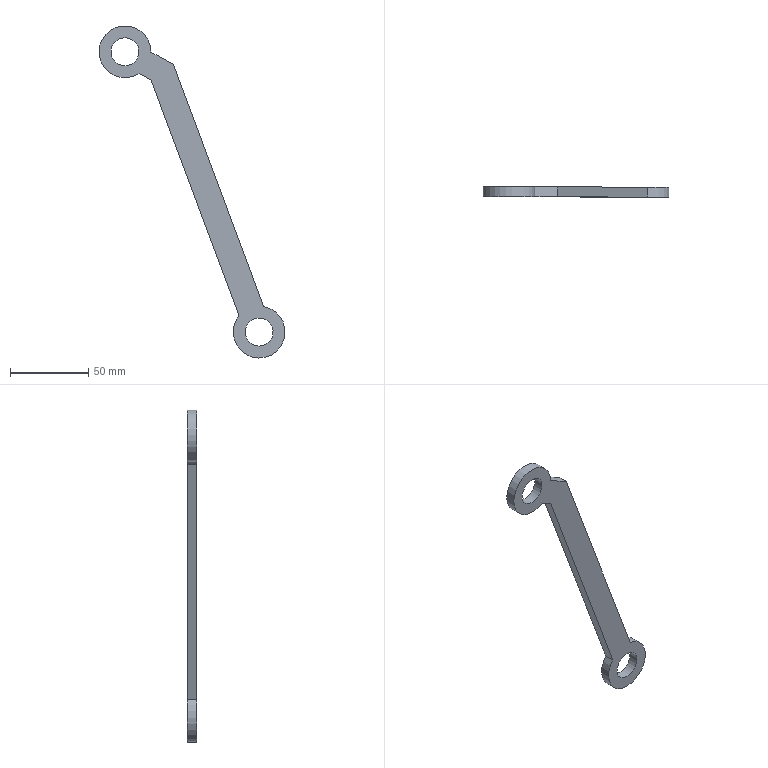Component | NX | LINK | 1 solid | 10 faces | box 118.49 x 6.35 x 211.58 mm | volume 25994 mm3 | plane 6 | cylinder 4 | commonest cylinder face diameters 33.02 x2 17.78 x2
STEP:
#1=CARTESIAN_POINT('',(0.,0.,0.));
#2=DIRECTION('',(0.,0.,1.));
#3=DIRECTION('',(1.,0.,0.));
#4=AXIS2_PLACEMENT_3D('',#1,#2,#3);
#5=CARTESIAN_POINT('',(88.37,21.5,328.882));
#6=VERTEX_POINT('',#5);
#7=CARTESIAN_POINT('',(72.634,21.5,323.014));
#8=VERTEX_POINT('',#7);
#9=CARTESIAN_POINT('',(85.469,21.5,312.629));
#10=DIRECTION('',(0.,1.,0.));
#11=DIRECTION('',(0.937,0.,0.3494));
#12=AXIS2_PLACEMENT_3D('',#9,#10,#11);
#13=CIRCLE('',#12,16.51);
#14=CARTESIAN_POINT('',(85.469,15.15,312.629));
#15=DIRECTION('',(0.,1.,0.));
#16=DIRECTION('',(-0.937,0.,-0.3494));
#17=AXIS2_PLACEMENT_3D('',#14,#15,#16);
#18=CYLINDRICAL_SURFACE('',#17,16.51);
#19=CARTESIAN_POINT('',(-3.142,6.35));
#20=DIRECTION('',(1.,0.));
#21=VECTOR('',#20,1.);
#22=LINE('',#19,#21);
#23=(GEOMETRIC_REPRESENTATION_CONTEXT(2)PARAMETRIC_REPRESENTATION_CONTEXT()REPRESENTATION_CONTEXT('',''));
#24=DEFINITIONAL_REPRESENTATION('',(#22),#23);
#25=PCURVE('',#18,#24);
#26=CARTESIAN_POINT('',(85.469,21.5,312.629));
#27=DIRECTION('',(0.,1.,0.));
#28=DIRECTION('',(-0.937,0.,-0.3494));
#29=AXIS2_PLACEMENT_3D('',#26,#27,#28);
#30=PLANE('',#29);
#31=CARTESIAN_POINT('',(0.,0.));
#32=DIRECTION('',(-1.,0.));
#33=AXIS2_PLACEMENT_2D('',#31,#32);
#34=CIRCLE('',#33,16.51);
#35=(GEOMETRIC_REPRESENTATION_CONTEXT(2)PARAMETRIC_REPRESENTATION_CONTEXT()REPRESENTATION_CONTEXT('',''));
#36=DEFINITIONAL_REPRESENTATION('',(#34),#35);
#37=PCURVE('',#30,#36);
#38=SURFACE_CURVE('',#13,(#25,#37),.PCURVE_S1.);
#39=EDGE_CURVE('',#6,#8,#38,.T.);
#40=ORIENTED_EDGE('',*,*,#39,.F.);
#41=CARTESIAN_POINT('',(88.37,15.15,328.882));
#42=VERTEX_POINT('',#41);
#43=CARTESIAN_POINT('',(88.37,15.15,328.882));
#44=DIRECTION('',(0.,1.,0.));
#45=VECTOR('',#44,1.);
#46=LINE('',#43,#45);
#47=CARTESIAN_POINT('',(2.104,0.));
#48=DIRECTION('',(0.,1.));
#49=VECTOR('',#48,1.);
#50=LINE('',#47,#49);
#51=(GEOMETRIC_REPRESENTATION_CONTEXT(2)PARAMETRIC_REPRESENTATION_CONTEXT()REPRESENTATION_CONTEXT('',''));
#52=DEFINITIONAL_REPRESENTATION('',(#50),#51);
#53=PCURVE('',#18,#52);
#54=CARTESIAN_POINT('',(30.849,15.15,483.124));
#55=DIRECTION('',(0.937,0.,0.3494));
#56=DIRECTION('',(-0.3494,0.,0.937));
#57=AXIS2_PLACEMENT_3D('',#54,#55,#56);
#58=PLANE('',#57);
#59=CARTESIAN_POINT('',(-164.619,0.));
#60=DIRECTION('',(0.,-1.));
#61=VECTOR('',#60,1.);
#62=LINE('',#59,#61);
#63=(GEOMETRIC_REPRESENTATION_CONTEXT(2)PARAMETRIC_REPRESENTATION_CONTEXT()REPRESENTATION_CONTEXT('',''));
#64=DEFINITIONAL_REPRESENTATION('',(#62),#63);
#65=PCURVE('',#58,#64);
#66=SURFACE_CURVE('',#46,(#53,#65),.PCURVE_S1.);
#67=EDGE_CURVE('',#42,#6,#66,.T.);
#68=ORIENTED_EDGE('',*,*,#67,.F.);
#69=CARTESIAN_POINT('',(72.634,15.15,323.014));
#70=VERTEX_POINT('',#69);
#71=CARTESIAN_POINT('',(85.469,15.15,312.629));
#72=DIRECTION('',(0.,1.,0.));
#73=DIRECTION('',(0.937,0.,0.3494));
#74=AXIS2_PLACEMENT_3D('',#71,#72,#73);
#75=CIRCLE('',#74,16.51);
#76=CARTESIAN_POINT('',(-3.142,0.));
#77=DIRECTION('',(1.,0.));
#78=VECTOR('',#77,1.);
#79=LINE('',#76,#78);
#80=(GEOMETRIC_REPRESENTATION_CONTEXT(2)PARAMETRIC_REPRESENTATION_CONTEXT()REPRESENTATION_CONTEXT('',''));
#81=DEFINITIONAL_REPRESENTATION('',(#79),#80);
#82=PCURVE('',#18,#81);
#83=CARTESIAN_POINT('',(85.469,15.15,312.629));
#84=DIRECTION('',(0.,1.,0.));
#85=DIRECTION('',(-0.937,0.,-0.3494));
#86=AXIS2_PLACEMENT_3D('',#83,#84,#85);
#87=PLANE('',#86);
#88=CARTESIAN_POINT('',(0.,0.));
#89=DIRECTION('',(-1.,0.));
#90=AXIS2_PLACEMENT_2D('',#88,#89);
#91=CIRCLE('',#90,16.51);
#92=(GEOMETRIC_REPRESENTATION_CONTEXT(2)PARAMETRIC_REPRESENTATION_CONTEXT()REPRESENTATION_CONTEXT('',''));
#93=DEFINITIONAL_REPRESENTATION('',(#91),#92);
#94=PCURVE('',#87,#93);
#95=SURFACE_CURVE('',#75,(#82,#94),.PCURVE_S1.);
#96=EDGE_CURVE('',#42,#70,#95,.T.);
#97=ORIENTED_EDGE('',*,*,#96,.T.);
#98=CARTESIAN_POINT('',(72.634,15.15,323.014));
#99=DIRECTION('',(0.,1.,0.));
#100=VECTOR('',#99,1.);
#101=LINE('',#98,#100);
#102=CARTESIAN_POINT('',(7.32,0.));
#103=DIRECTION('',(0.,1.));
#104=VECTOR('',#103,1.);
#105=LINE('',#102,#104);
#106=(GEOMETRIC_REPRESENTATION_CONTEXT(2)PARAMETRIC_REPRESENTATION_CONTEXT()REPRESENTATION_CONTEXT('',''));
#107=DEFINITIONAL_REPRESENTATION('',(#105),#106);
#108=PCURVE('',#18,#107);
#109=CARTESIAN_POINT('',(72.634,15.15,323.014));
#110=DIRECTION('',(-0.937,0.,-0.3494));
#111=DIRECTION('',(0.3494,0.,-0.937));
#112=AXIS2_PLACEMENT_3D('',#109,#110,#111);
#113=PLANE('',#112);
#114=CARTESIAN_POINT('',(0.,0.));
#115=DIRECTION('',(0.,-1.));
#116=VECTOR('',#115,1.);
#117=LINE('',#114,#116);
#118=(GEOMETRIC_REPRESENTATION_CONTEXT(2)PARAMETRIC_REPRESENTATION_CONTEXT()REPRESENTATION_CONTEXT('',''));
#119=DEFINITIONAL_REPRESENTATION('',(#117),#118);
#120=PCURVE('',#113,#119);
#121=SURFACE_CURVE('',#101,(#108,#120),.PCURVE_S1.);
#122=EDGE_CURVE('',#70,#8,#121,.T.);
#123=ORIENTED_EDGE('',*,*,#122,.T.);
#124=EDGE_LOOP('',(#40,#68,#97,#123));
#125=FACE_BOUND('',#124,.T.);
#126=ADVANCED_FACE('',(#125),#18,.T.);
#127=CARTESIAN_POINT('',(16.679,21.5,473.058));
#128=VERTEX_POINT('',#127);
#129=CARTESIAN_POINT('',(72.634,21.5,323.014));
#130=DIRECTION('',(-0.3494,0.,0.937));
#131=VECTOR('',#130,1.);
#132=LINE('',#129,#131);
#133=CARTESIAN_POINT('',(0.,-6.35));
#134=DIRECTION('',(-1.,0.));
#135=VECTOR('',#134,1.);
#136=LINE('',#133,#135);
#137=(GEOMETRIC_REPRESENTATION_CONTEXT(2)PARAMETRIC_REPRESENTATION_CONTEXT()REPRESENTATION_CONTEXT('',''));
#138=DEFINITIONAL_REPRESENTATION('',(#136),#137);
#139=PCURVE('',#113,#138);
#140=CARTESIAN_POINT('',(8.397,14.215));
#141=DIRECTION('',(0.,1.));
#142=VECTOR('',#141,1.);
#143=LINE('',#140,#142);
#144=(GEOMETRIC_REPRESENTATION_CONTEXT(2)PARAMETRIC_REPRESENTATION_CONTEXT()REPRESENTATION_CONTEXT('',''));
#145=DEFINITIONAL_REPRESENTATION('',(#143),#144);
#146=PCURVE('',#30,#145);
#147=SURFACE_CURVE('',#132,(#139,#146),.PCURVE_S1.);
#148=EDGE_CURVE('',#8,#128,#147,.T.);
#149=ORIENTED_EDGE('',*,*,#148,.F.);
#150=ORIENTED_EDGE('',*,*,#122,.F.);
#151=CARTESIAN_POINT('',(16.679,15.15,473.058));
#152=VERTEX_POINT('',#151);
#153=CARTESIAN_POINT('',(72.634,15.15,323.014));
#154=DIRECTION('',(-0.3494,0.,0.937));
#155=VECTOR('',#154,1.);
#156=LINE('',#153,#155);
#157=CARTESIAN_POINT('',(0.,0.));
#158=DIRECTION('',(-1.,0.));
#159=VECTOR('',#158,1.);
#160=LINE('',#157,#159);
#161=(GEOMETRIC_REPRESENTATION_CONTEXT(2)PARAMETRIC_REPRESENTATION_CONTEXT()REPRESENTATION_CONTEXT('',''));
#162=DEFINITIONAL_REPRESENTATION('',(#160),#161);
#163=PCURVE('',#113,#162);
#164=CARTESIAN_POINT('',(8.397,14.215));
#165=DIRECTION('',(0.,1.));
#166=VECTOR('',#165,1.);
#167=LINE('',#164,#166);
#168=(GEOMETRIC_REPRESENTATION_CONTEXT(2)PARAMETRIC_REPRESENTATION_CONTEXT()REPRESENTATION_CONTEXT('',''));
#169=DEFINITIONAL_REPRESENTATION('',(#167),#168);
#170=PCURVE('',#87,#169);
#171=SURFACE_CURVE('',#156,(#163,#170),.PCURVE_S1.);
#172=EDGE_CURVE('',#70,#152,#171,.T.);
#173=ORIENTED_EDGE('',*,*,#172,.T.);
#174=CARTESIAN_POINT('',(16.679,15.15,473.058));
#175=DIRECTION('',(0.,1.,0.));
#176=VECTOR('',#175,1.);
#177=LINE('',#174,#176);
#178=CARTESIAN_POINT('',(-160.139,0.));
#179=DIRECTION('',(0.,-1.));
#180=VECTOR('',#179,1.);
#181=LINE('',#178,#180);
#182=(GEOMETRIC_REPRESENTATION_CONTEXT(2)PARAMETRIC_REPRESENTATION_CONTEXT()REPRESENTATION_CONTEXT('',''));
#183=DEFINITIONAL_REPRESENTATION('',(#181),#182);
#184=PCURVE('',#113,#183);
#185=CARTESIAN_POINT('',(16.679,15.15,473.058));
#186=DIRECTION('',(-0.4827,0.,-0.8758));
#187=DIRECTION('',(0.8758,0.,-0.4827));
#188=AXIS2_PLACEMENT_3D('',#185,#186,#187);
#189=PLANE('',#188);
#190=CARTESIAN_POINT('',(0.,0.));
#191=DIRECTION('',(0.,-1.));
#192=VECTOR('',#191,1.);
#193=LINE('',#190,#192);
#194=(GEOMETRIC_REPRESENTATION_CONTEXT(2)PARAMETRIC_REPRESENTATION_CONTEXT()REPRESENTATION_CONTEXT('',''));
#195=DEFINITIONAL_REPRESENTATION('',(#193),#194);
#196=PCURVE('',#189,#195);
#197=SURFACE_CURVE('',#177,(#184,#196),.PCURVE_S1.);
#198=EDGE_CURVE('',#152,#128,#197,.T.);
#199=ORIENTED_EDGE('',*,*,#198,.T.);
#200=EDGE_LOOP('',(#149,#150,#173,#199));
#201=FACE_BOUND('',#200,.T.);
#202=ADVANCED_FACE('',(#201),#113,.T.);
#203=CARTESIAN_POINT('',(8.952,21.5,477.318));
#204=VERTEX_POINT('',#203);
#205=CARTESIAN_POINT('',(16.679,21.5,473.058));
#206=DIRECTION('',(-0.8758,0.,0.4827));
#207=VECTOR('',#206,1.);
#208=LINE('',#205,#207);
#209=CARTESIAN_POINT('',(0.,-6.35));
#210=DIRECTION('',(-1.,0.));
#211=VECTOR('',#210,1.);
#212=LINE('',#209,#211);
#213=(GEOMETRIC_REPRESENTATION_CONTEXT(2)PARAMETRIC_REPRESENTATION_CONTEXT()REPRESENTATION_CONTEXT('',''));
#214=DEFINITIONAL_REPRESENTATION('',(#212),#213);
#215=PCURVE('',#189,#214);
#216=CARTESIAN_POINT('',(8.397,174.354));
#217=DIRECTION('',(0.6519,0.7583));
#218=VECTOR('',#217,1.);
#219=LINE('',#216,#218);
#220=(GEOMETRIC_REPRESENTATION_CONTEXT(2)PARAMETRIC_REPRESENTATION_CONTEXT()REPRESENTATION_CONTEXT('',''));
#221=DEFINITIONAL_REPRESENTATION('',(#219),#220);
#222=PCURVE('',#30,#221);
#223=SURFACE_CURVE('',#208,(#215,#222),.PCURVE_S1.);
#224=EDGE_CURVE('',#128,#204,#223,.T.);
#225=ORIENTED_EDGE('',*,*,#224,.F.);
#226=ORIENTED_EDGE('',*,*,#198,.F.);
#227=CARTESIAN_POINT('',(8.952,15.15,477.318));
#228=VERTEX_POINT('',#227);
#229=CARTESIAN_POINT('',(16.679,15.15,473.058));
#230=DIRECTION('',(-0.8758,0.,0.4827));
#231=VECTOR('',#230,1.);
#232=LINE('',#229,#231);
#233=CARTESIAN_POINT('',(0.,0.));
#234=DIRECTION('',(-1.,0.));
#235=VECTOR('',#234,1.);
#236=LINE('',#233,#235);
#237=(GEOMETRIC_REPRESENTATION_CONTEXT(2)PARAMETRIC_REPRESENTATION_CONTEXT()REPRESENTATION_CONTEXT('',''));
#238=DEFINITIONAL_REPRESENTATION('',(#236),#237);
#239=PCURVE('',#189,#238);
#240=CARTESIAN_POINT('',(8.397,174.354));
#241=DIRECTION('',(0.6519,0.7583));
#242=VECTOR('',#241,1.);
#243=LINE('',#240,#242);
#244=(GEOMETRIC_REPRESENTATION_CONTEXT(2)PARAMETRIC_REPRESENTATION_CONTEXT()REPRESENTATION_CONTEXT('',''));
#245=DEFINITIONAL_REPRESENTATION('',(#243),#244);
#246=PCURVE('',#87,#245);
#247=SURFACE_CURVE('',#232,(#239,#246),.PCURVE_S1.);
#248=EDGE_CURVE('',#152,#228,#247,.T.);
#249=ORIENTED_EDGE('',*,*,#248,.T.);
#250=CARTESIAN_POINT('',(8.952,15.15,477.318));
#251=DIRECTION('',(0.,1.,0.));
#252=VECTOR('',#251,1.);
#253=LINE('',#250,#252);
#254=CARTESIAN_POINT('',(-8.823,0.));
#255=DIRECTION('',(0.,-1.));
#256=VECTOR('',#255,1.);
#257=LINE('',#254,#256);
#258=(GEOMETRIC_REPRESENTATION_CONTEXT(2)PARAMETRIC_REPRESENTATION_CONTEXT()REPRESENTATION_CONTEXT('',''));
#259=DEFINITIONAL_REPRESENTATION('',(#257),#258);
#260=PCURVE('',#189,#259);
#261=CARTESIAN_POINT('',(0.,15.15,491.19));
#262=DIRECTION('',(0.,1.,0.));
#263=DIRECTION('',(-0.937,0.,-0.3494));
#264=AXIS2_PLACEMENT_3D('',#261,#262,#263);
#265=CYLINDRICAL_SURFACE('',#264,16.51);
#266=CARTESIAN_POINT('',(-1.787,0.));
#267=DIRECTION('',(0.,1.));
#268=VECTOR('',#267,1.);
#269=LINE('',#266,#268);
#270=(GEOMETRIC_REPRESENTATION_CONTEXT(2)PARAMETRIC_REPRESENTATION_CONTEXT()REPRESENTATION_CONTEXT('',''));
#271=DEFINITIONAL_REPRESENTATION('',(#269),#270);
#272=PCURVE('',#265,#271);
#273=SURFACE_CURVE('',#253,(#260,#272),.PCURVE_S1.);
#274=EDGE_CURVE('',#228,#204,#273,.T.);
#275=ORIENTED_EDGE('',*,*,#274,.T.);
#276=EDGE_LOOP('',(#225,#226,#249,#275));
#277=FACE_BOUND('',#276,.T.);
#278=ADVANCED_FACE('',(#277),#189,.T.);
#279=CARTESIAN_POINT('',(16.509,21.5,491.028));
#280=VERTEX_POINT('',#279);
#281=CARTESIAN_POINT('',(0.,21.5,491.19));
#282=DIRECTION('',(0.,1.,0.));
#283=DIRECTION('',(0.937,0.,0.3494));
#284=AXIS2_PLACEMENT_3D('',#281,#282,#283);
#285=CIRCLE('',#284,16.51);
#286=CARTESIAN_POINT('',(-3.142,6.35));
#287=DIRECTION('',(1.,0.));
#288=VECTOR('',#287,1.);
#289=LINE('',#286,#288);
#290=(GEOMETRIC_REPRESENTATION_CONTEXT(2)PARAMETRIC_REPRESENTATION_CONTEXT()REPRESENTATION_CONTEXT('',''));
#291=DEFINITIONAL_REPRESENTATION('',(#289),#290);
#292=PCURVE('',#265,#291);
#293=CARTESIAN_POINT('',(17.689,197.171));
#294=DIRECTION('',(-1.,0.));
#295=AXIS2_PLACEMENT_2D('',#293,#294);
#296=CIRCLE('',#295,16.51);
#297=(GEOMETRIC_REPRESENTATION_CONTEXT(2)PARAMETRIC_REPRESENTATION_CONTEXT()REPRESENTATION_CONTEXT('',''));
#298=DEFINITIONAL_REPRESENTATION('',(#296),#297);
#299=PCURVE('',#30,#298);
#300=SURFACE_CURVE('',#285,(#292,#299),.PCURVE_S1.);
#301=EDGE_CURVE('',#204,#280,#300,.T.);
#302=ORIENTED_EDGE('',*,*,#301,.F.);
#303=ORIENTED_EDGE('',*,*,#274,.F.);
#304=CARTESIAN_POINT('',(16.509,15.15,491.028));
#305=VERTEX_POINT('',#304);
#306=CARTESIAN_POINT('',(0.,15.15,491.19));
#307=DIRECTION('',(0.,1.,0.));
#308=DIRECTION('',(0.937,0.,0.3494));
#309=AXIS2_PLACEMENT_3D('',#306,#307,#308);
#310=CIRCLE('',#309,16.51);
#311=CARTESIAN_POINT('',(-3.142,0.));
#312=DIRECTION('',(1.,0.));
#313=VECTOR('',#312,1.);
#314=LINE('',#311,#313);
#315=(GEOMETRIC_REPRESENTATION_CONTEXT(2)PARAMETRIC_REPRESENTATION_CONTEXT()REPRESENTATION_CONTEXT('',''));
#316=DEFINITIONAL_REPRESENTATION('',(#314),#315);
#317=PCURVE('',#265,#316);
#318=CARTESIAN_POINT('',(17.689,197.171));
#319=DIRECTION('',(-1.,0.));
#320=AXIS2_PLACEMENT_2D('',#318,#319);
#321=CIRCLE('',#320,16.51);
#322=(GEOMETRIC_REPRESENTATION_CONTEXT(2)PARAMETRIC_REPRESENTATION_CONTEXT()REPRESENTATION_CONTEXT('',''));
#323=DEFINITIONAL_REPRESENTATION('',(#321),#322);
#324=PCURVE('',#87,#323);
#325=SURFACE_CURVE('',#310,(#317,#324),.PCURVE_S1.);
#326=EDGE_CURVE('',#228,#305,#325,.T.);
#327=ORIENTED_EDGE('',*,*,#326,.T.);
#328=CARTESIAN_POINT('',(16.509,15.15,491.028));
#329=DIRECTION('',(0.,1.,0.));
#330=VECTOR('',#329,1.);
#331=LINE('',#328,#330);
#332=CARTESIAN_POINT('',(3.508,0.));
#333=DIRECTION('',(0.,1.));
#334=VECTOR('',#333,1.);
#335=LINE('',#332,#334);
#336=(GEOMETRIC_REPRESENTATION_CONTEXT(2)PARAMETRIC_REPRESENTATION_CONTEXT()REPRESENTATION_CONTEXT('',''));
#337=DEFINITIONAL_REPRESENTATION('',(#335),#336);
#338=PCURVE('',#265,#337);
#339=CARTESIAN_POINT('',(16.509,15.15,491.028));
#340=DIRECTION('',(0.4827,0.,0.8758));
#341=DIRECTION('',(-0.8758,0.,0.4827));
#342=AXIS2_PLACEMENT_3D('',#339,#340,#341);
#343=PLANE('',#342);
#344=CARTESIAN_POINT('',(0.,0.));
#345=DIRECTION('',(0.,-1.));
#346=VECTOR('',#345,1.);
#347=LINE('',#344,#346);
#348=(GEOMETRIC_REPRESENTATION_CONTEXT(2)PARAMETRIC_REPRESENTATION_CONTEXT()REPRESENTATION_CONTEXT('',''));
#349=DEFINITIONAL_REPRESENTATION('',(#347),#348);
#350=PCURVE('',#343,#349);
#351=SURFACE_CURVE('',#331,(#338,#350),.PCURVE_S1.);
#352=EDGE_CURVE('',#305,#280,#351,.T.);
#353=ORIENTED_EDGE('',*,*,#352,.T.);
#354=EDGE_LOOP('',(#302,#303,#327,#353));
#355=FACE_BOUND('',#354,.T.);
#356=ADVANCED_FACE('',(#355),#265,.T.);
#357=CARTESIAN_POINT('',(30.849,21.5,483.124));
#358=VERTEX_POINT('',#357);
#359=CARTESIAN_POINT('',(16.509,21.5,491.028));
#360=DIRECTION('',(0.8758,0.,-0.4827));
#361=VECTOR('',#360,1.);
#362=LINE('',#359,#361);
#363=CARTESIAN_POINT('',(0.,-6.35));
#364=DIRECTION('',(-1.,0.));
#365=VECTOR('',#364,1.);
#366=LINE('',#363,#365);
#367=(GEOMETRIC_REPRESENTATION_CONTEXT(2)PARAMETRIC_REPRESENTATION_CONTEXT()REPRESENTATION_CONTEXT('',''));
#368=DEFINITIONAL_REPRESENTATION('',(#366),#367);
#369=PCURVE('',#343,#368);
#370=CARTESIAN_POINT('',(2.277,191.251));
#371=DIRECTION('',(-0.6519,-0.7583));
#372=VECTOR('',#371,1.);
#373=LINE('',#370,#372);
#374=(GEOMETRIC_REPRESENTATION_CONTEXT(2)PARAMETRIC_REPRESENTATION_CONTEXT()REPRESENTATION_CONTEXT('',''));
#375=DEFINITIONAL_REPRESENTATION('',(#373),#374);
#376=PCURVE('',#30,#375);
#377=SURFACE_CURVE('',#362,(#369,#376),.PCURVE_S1.);
#378=EDGE_CURVE('',#280,#358,#377,.T.);
#379=ORIENTED_EDGE('',*,*,#378,.F.);
#380=ORIENTED_EDGE('',*,*,#352,.F.);
#381=CARTESIAN_POINT('',(30.849,15.15,483.124));
#382=VERTEX_POINT('',#381);
#383=CARTESIAN_POINT('',(16.509,15.15,491.028));
#384=DIRECTION('',(0.8758,0.,-0.4827));
#385=VECTOR('',#384,1.);
#386=LINE('',#383,#385);
#387=CARTESIAN_POINT('',(0.,0.));
#388=DIRECTION('',(-1.,0.));
#389=VECTOR('',#388,1.);
#390=LINE('',#387,#389);
#391=(GEOMETRIC_REPRESENTATION_CONTEXT(2)PARAMETRIC_REPRESENTATION_CONTEXT()REPRESENTATION_CONTEXT('',''));
#392=DEFINITIONAL_REPRESENTATION('',(#390),#391);
#393=PCURVE('',#343,#392);
#394=CARTESIAN_POINT('',(2.277,191.251));
#395=DIRECTION('',(-0.6519,-0.7583));
#396=VECTOR('',#395,1.);
#397=LINE('',#394,#396);
#398=(GEOMETRIC_REPRESENTATION_CONTEXT(2)PARAMETRIC_REPRESENTATION_CONTEXT()REPRESENTATION_CONTEXT('',''));
#399=DEFINITIONAL_REPRESENTATION('',(#397),#398);
#400=PCURVE('',#87,#399);
#401=SURFACE_CURVE('',#386,(#393,#400),.PCURVE_S1.);
#402=EDGE_CURVE('',#305,#382,#401,.T.);
#403=ORIENTED_EDGE('',*,*,#402,.T.);
#404=CARTESIAN_POINT('',(30.849,15.15,483.124));
#405=DIRECTION('',(0.,1.,0.));
#406=VECTOR('',#405,1.);
#407=LINE('',#404,#406);
#408=CARTESIAN_POINT('',(-16.374,0.));
#409=DIRECTION('',(0.,-1.));
#410=VECTOR('',#409,1.);
#411=LINE('',#408,#410);
#412=(GEOMETRIC_REPRESENTATION_CONTEXT(2)PARAMETRIC_REPRESENTATION_CONTEXT()REPRESENTATION_CONTEXT('',''));
#413=DEFINITIONAL_REPRESENTATION('',(#411),#412);
#414=PCURVE('',#343,#413);
#415=CARTESIAN_POINT('',(0.,0.));
#416=DIRECTION('',(0.,-1.));
#417=VECTOR('',#416,1.);
#418=LINE('',#415,#417);
#419=(GEOMETRIC_REPRESENTATION_CONTEXT(2)PARAMETRIC_REPRESENTATION_CONTEXT()REPRESENTATION_CONTEXT('',''));
#420=DEFINITIONAL_REPRESENTATION('',(#418),#419);
#421=PCURVE('',#58,#420);
#422=SURFACE_CURVE('',#407,(#414,#421),.PCURVE_S1.);
#423=EDGE_CURVE('',#382,#358,#422,.T.);
#424=ORIENTED_EDGE('',*,*,#423,.T.);
#425=EDGE_LOOP('',(#379,#380,#403,#424));
#426=FACE_BOUND('',#425,.T.);
#427=ADVANCED_FACE('',(#426),#343,.T.);
#428=CARTESIAN_POINT('',(93.799,15.15,315.735));
#429=VERTEX_POINT('',#428);
#430=CARTESIAN_POINT('',(85.469,15.15,312.629));
#431=DIRECTION('',(0.,1.,0.));
#432=DIRECTION('',(0.937,0.,0.3494));
#433=AXIS2_PLACEMENT_3D('',#430,#431,#432);
#434=CIRCLE('',#433,8.89);
#435=CARTESIAN_POINT('',(85.469,15.15,312.629));
#436=DIRECTION('',(0.,1.,0.));
#437=DIRECTION('',(-0.937,0.,-0.3494));
#438=AXIS2_PLACEMENT_3D('',#435,#436,#437);
#439=CYLINDRICAL_SURFACE('',#438,8.89);
#440=CARTESIAN_POINT('',(3.142,0.));
#441=DIRECTION('',(1.,0.));
#442=VECTOR('',#441,1.);
#443=LINE('',#440,#442);
#444=(GEOMETRIC_REPRESENTATION_CONTEXT(2)PARAMETRIC_REPRESENTATION_CONTEXT()REPRESENTATION_CONTEXT('',''));
#445=DEFINITIONAL_REPRESENTATION('',(#443),#444);
#446=PCURVE('',#439,#445);
#447=CARTESIAN_POINT('',(0.,0.));
#448=DIRECTION('',(-1.,0.));
#449=AXIS2_PLACEMENT_2D('',#447,#448);
#450=CIRCLE('',#449,8.89);
#451=(GEOMETRIC_REPRESENTATION_CONTEXT(2)PARAMETRIC_REPRESENTATION_CONTEXT()REPRESENTATION_CONTEXT('',''));
#452=DEFINITIONAL_REPRESENTATION('',(#450),#451);
#453=PCURVE('',#87,#452);
#454=SURFACE_CURVE('',#434,(#446,#453),.PCURVE_S1.);
#455=EDGE_CURVE('',#429,#429,#454,.T.);
#456=ORIENTED_EDGE('',*,*,#455,.T.);
#457=CARTESIAN_POINT('',(93.799,21.5,315.735));
#458=VERTEX_POINT('',#457);
#459=CARTESIAN_POINT('',(93.799,15.15,315.735));
#460=CARTESIAN_POINT('',(93.799,21.5,315.735));
#461=B_SPLINE_CURVE_WITH_KNOTS('',1,(#459,#460),.UNSPECIFIED.,.F.,.F.,(2,2),(0.,6.35),.PIECEWISE_BEZIER_KNOTS.);
#462=CARTESIAN_POINT('',(9.425,0.));
#463=DIRECTION('',(0.,1.));
#464=VECTOR('',#463,1.);
#465=LINE('',#462,#464);
#466=(GEOMETRIC_REPRESENTATION_CONTEXT(2)PARAMETRIC_REPRESENTATION_CONTEXT()REPRESENTATION_CONTEXT('',''));
#467=DEFINITIONAL_REPRESENTATION('',(#465),#466);
#468=PCURVE('',#439,#467);
#469=CARTESIAN_POINT('',(3.142,0.));
#470=DIRECTION('',(0.,1.));
#471=VECTOR('',#470,1.);
#472=LINE('',#469,#471);
#473=(GEOMETRIC_REPRESENTATION_CONTEXT(2)PARAMETRIC_REPRESENTATION_CONTEXT()REPRESENTATION_CONTEXT('',''));
#474=DEFINITIONAL_REPRESENTATION('',(#472),#473);
#475=PCURVE('',#439,#474);
#476=SEAM_CURVE('',#461,(#468,#475),.PCURVE_S1.);
#477=EDGE_CURVE('',#429,#458,#476,.T.);
#478=ORIENTED_EDGE('',*,*,#477,.T.);
#479=CARTESIAN_POINT('',(85.469,21.5,312.629));
#480=DIRECTION('',(0.,1.,0.));
#481=DIRECTION('',(0.937,0.,0.3494));
#482=AXIS2_PLACEMENT_3D('',#479,#480,#481);
#483=CIRCLE('',#482,8.89);
#484=CARTESIAN_POINT('',(3.142,6.35));
#485=DIRECTION('',(1.,0.));
#486=VECTOR('',#485,1.);
#487=LINE('',#484,#486);
#488=(GEOMETRIC_REPRESENTATION_CONTEXT(2)PARAMETRIC_REPRESENTATION_CONTEXT()REPRESENTATION_CONTEXT('',''));
#489=DEFINITIONAL_REPRESENTATION('',(#487),#488);
#490=PCURVE('',#439,#489);
#491=CARTESIAN_POINT('',(0.,0.));
#492=DIRECTION('',(-1.,0.));
#493=AXIS2_PLACEMENT_2D('',#491,#492);
#494=CIRCLE('',#493,8.89);
#495=(GEOMETRIC_REPRESENTATION_CONTEXT(2)PARAMETRIC_REPRESENTATION_CONTEXT()REPRESENTATION_CONTEXT('',''));
#496=DEFINITIONAL_REPRESENTATION('',(#494),#495);
#497=PCURVE('',#30,#496);
#498=SURFACE_CURVE('',#483,(#490,#497),.PCURVE_S1.);
#499=EDGE_CURVE('',#458,#458,#498,.T.);
#500=ORIENTED_EDGE('',*,*,#499,.F.);
#501=ORIENTED_EDGE('',*,*,#477,.F.);
#502=EDGE_LOOP('',(#456,#478,#500,#501));
#503=FACE_BOUND('',#502,.F.);
#504=ADVANCED_FACE('',(#503),#439,.F.);
#505=CARTESIAN_POINT('',(30.849,21.5,483.124));
#506=DIRECTION('',(0.3494,0.,-0.937));
#507=VECTOR('',#506,1.);
#508=LINE('',#505,#507);
#509=CARTESIAN_POINT('',(0.,-6.35));
#510=DIRECTION('',(-1.,0.));
#511=VECTOR('',#510,1.);
#512=LINE('',#509,#511);
#513=(GEOMETRIC_REPRESENTATION_CONTEXT(2)PARAMETRIC_REPRESENTATION_CONTEXT()REPRESENTATION_CONTEXT('',''));
#514=DEFINITIONAL_REPRESENTATION('',(#512),#513);
#515=PCURVE('',#58,#514);
#516=CARTESIAN_POINT('',(-8.397,178.834));
#517=DIRECTION('',(0.,-1.));
#518=VECTOR('',#517,1.);
#519=LINE('',#516,#518);
#520=(GEOMETRIC_REPRESENTATION_CONTEXT(2)PARAMETRIC_REPRESENTATION_CONTEXT()REPRESENTATION_CONTEXT('',''));
#521=DEFINITIONAL_REPRESENTATION('',(#519),#520);
#522=PCURVE('',#30,#521);
#523=SURFACE_CURVE('',#508,(#515,#522),.PCURVE_S1.);
#524=EDGE_CURVE('',#358,#6,#523,.T.);
#525=ORIENTED_EDGE('',*,*,#524,.F.);
#526=ORIENTED_EDGE('',*,*,#423,.F.);
#527=CARTESIAN_POINT('',(30.849,15.15,483.124));
#528=DIRECTION('',(0.3494,0.,-0.937));
#529=VECTOR('',#528,1.);
#530=LINE('',#527,#529);
#531=CARTESIAN_POINT('',(0.,0.));
#532=DIRECTION('',(-1.,0.));
#533=VECTOR('',#532,1.);
#534=LINE('',#531,#533);
#535=(GEOMETRIC_REPRESENTATION_CONTEXT(2)PARAMETRIC_REPRESENTATION_CONTEXT()REPRESENTATION_CONTEXT('',''));
#536=DEFINITIONAL_REPRESENTATION('',(#534),#535);
#537=PCURVE('',#58,#536);
#538=CARTESIAN_POINT('',(-8.397,178.834));
#539=DIRECTION('',(0.,-1.));
#540=VECTOR('',#539,1.);
#541=LINE('',#538,#540);
#542=(GEOMETRIC_REPRESENTATION_CONTEXT(2)PARAMETRIC_REPRESENTATION_CONTEXT()REPRESENTATION_CONTEXT('',''));
#543=DEFINITIONAL_REPRESENTATION('',(#541),#542);
#544=PCURVE('',#87,#543);
#545=SURFACE_CURVE('',#530,(#537,#544),.PCURVE_S1.);
#546=EDGE_CURVE('',#382,#42,#545,.T.);
#547=ORIENTED_EDGE('',*,*,#546,.T.);
#548=ORIENTED_EDGE('',*,*,#67,.T.);
#549=EDGE_LOOP('',(#525,#526,#547,#548));
#550=FACE_BOUND('',#549,.T.);
#551=ADVANCED_FACE('',(#550),#58,.T.);
#552=CARTESIAN_POINT('',(8.33,15.15,494.296));
#553=VERTEX_POINT('',#552);
#554=CARTESIAN_POINT('',(0.,15.15,491.19));
#555=DIRECTION('',(0.,1.,0.));
#556=DIRECTION('',(0.937,0.,0.3494));
#557=AXIS2_PLACEMENT_3D('',#554,#555,#556);
#558=CIRCLE('',#557,8.89);
#559=CARTESIAN_POINT('',(0.,15.15,491.19));
#560=DIRECTION('',(0.,1.,0.));
#561=DIRECTION('',(-0.937,0.,-0.3494));
#562=AXIS2_PLACEMENT_3D('',#559,#560,#561);
#563=CYLINDRICAL_SURFACE('',#562,8.89);
#564=CARTESIAN_POINT('',(3.142,0.));
#565=DIRECTION('',(1.,0.));
#566=VECTOR('',#565,1.);
#567=LINE('',#564,#566);
#568=(GEOMETRIC_REPRESENTATION_CONTEXT(2)PARAMETRIC_REPRESENTATION_CONTEXT()REPRESENTATION_CONTEXT('',''));
#569=DEFINITIONAL_REPRESENTATION('',(#567),#568);
#570=PCURVE('',#563,#569);
#571=CARTESIAN_POINT('',(17.689,197.171));
#572=DIRECTION('',(-1.,0.));
#573=AXIS2_PLACEMENT_2D('',#571,#572);
#574=CIRCLE('',#573,8.89);
#575=(GEOMETRIC_REPRESENTATION_CONTEXT(2)PARAMETRIC_REPRESENTATION_CONTEXT()REPRESENTATION_CONTEXT('',''));
#576=DEFINITIONAL_REPRESENTATION('',(#574),#575);
#577=PCURVE('',#87,#576);
#578=SURFACE_CURVE('',#558,(#570,#577),.PCURVE_S1.);
#579=EDGE_CURVE('',#553,#553,#578,.T.);
#580=ORIENTED_EDGE('',*,*,#579,.T.);
#581=CARTESIAN_POINT('',(8.33,21.5,494.296));
#582=VERTEX_POINT('',#581);
#583=CARTESIAN_POINT('',(8.33,15.15,494.296));
#584=CARTESIAN_POINT('',(8.33,21.5,494.296));
#585=B_SPLINE_CURVE_WITH_KNOTS('',1,(#583,#584),.UNSPECIFIED.,.F.,.F.,(2,2),(0.,6.35),.PIECEWISE_BEZIER_KNOTS.);
#586=CARTESIAN_POINT('',(9.425,0.));
#587=DIRECTION('',(0.,1.));
#588=VECTOR('',#587,1.);
#589=LINE('',#586,#588);
#590=(GEOMETRIC_REPRESENTATION_CONTEXT(2)PARAMETRIC_REPRESENTATION_CONTEXT()REPRESENTATION_CONTEXT('',''));
#591=DEFINITIONAL_REPRESENTATION('',(#589),#590);
#592=PCURVE('',#563,#591);
#593=CARTESIAN_POINT('',(3.142,0.));
#594=DIRECTION('',(0.,1.));
#595=VECTOR('',#594,1.);
#596=LINE('',#593,#595);
#597=(GEOMETRIC_REPRESENTATION_CONTEXT(2)PARAMETRIC_REPRESENTATION_CONTEXT()REPRESENTATION_CONTEXT('',''));
#598=DEFINITIONAL_REPRESENTATION('',(#596),#597);
#599=PCURVE('',#563,#598);
#600=SEAM_CURVE('',#585,(#592,#599),.PCURVE_S1.);
#601=EDGE_CURVE('',#553,#582,#600,.T.);
#602=ORIENTED_EDGE('',*,*,#601,.T.);
#603=CARTESIAN_POINT('',(0.,21.5,491.19));
#604=DIRECTION('',(0.,1.,0.));
#605=DIRECTION('',(0.937,0.,0.3494));
#606=AXIS2_PLACEMENT_3D('',#603,#604,#605);
#607=CIRCLE('',#606,8.89);
#608=CARTESIAN_POINT('',(3.142,6.35));
#609=DIRECTION('',(1.,0.));
#610=VECTOR('',#609,1.);
#611=LINE('',#608,#610);
#612=(GEOMETRIC_REPRESENTATION_CONTEXT(2)PARAMETRIC_REPRESENTATION_CONTEXT()REPRESENTATION_CONTEXT('',''));
#613=DEFINITIONAL_REPRESENTATION('',(#611),#612);
#614=PCURVE('',#563,#613);
#615=CARTESIAN_POINT('',(17.689,197.171));
#616=DIRECTION('',(-1.,0.));
#617=AXIS2_PLACEMENT_2D('',#615,#616);
#618=CIRCLE('',#617,8.89);
#619=(GEOMETRIC_REPRESENTATION_CONTEXT(2)PARAMETRIC_REPRESENTATION_CONTEXT()REPRESENTATION_CONTEXT('',''));
#620=DEFINITIONAL_REPRESENTATION('',(#618),#619);
#621=PCURVE('',#30,#620);
#622=SURFACE_CURVE('',#607,(#614,#621),.PCURVE_S1.);
#623=EDGE_CURVE('',#582,#582,#622,.T.);
#624=ORIENTED_EDGE('',*,*,#623,.F.);
#625=ORIENTED_EDGE('',*,*,#601,.F.);
#626=EDGE_LOOP('',(#580,#602,#624,#625));
#627=FACE_BOUND('',#626,.F.);
#628=ADVANCED_FACE('',(#627),#563,.F.);
#629=ORIENTED_EDGE('',*,*,#96,.F.);
#630=ORIENTED_EDGE('',*,*,#546,.F.);
#631=ORIENTED_EDGE('',*,*,#402,.F.);
#632=ORIENTED_EDGE('',*,*,#326,.F.);
#633=ORIENTED_EDGE('',*,*,#248,.F.);
#634=ORIENTED_EDGE('',*,*,#172,.F.);
#635=EDGE_LOOP('',(#629,#630,#631,#632,#633,#634));
#636=FACE_BOUND('',#635,.T.);
#637=ORIENTED_EDGE('',*,*,#455,.T.);
#638=EDGE_LOOP('',(#637));
#639=FACE_BOUND('',#638,.T.);
#640=ORIENTED_EDGE('',*,*,#579,.T.);
#641=EDGE_LOOP('',(#640));
#642=FACE_BOUND('',#641,.T.);
#643=ADVANCED_FACE('',(#636,#639,#642),#87,.F.);
#644=ORIENTED_EDGE('',*,*,#39,.T.);
#645=ORIENTED_EDGE('',*,*,#148,.T.);
#646=ORIENTED_EDGE('',*,*,#224,.T.);
#647=ORIENTED_EDGE('',*,*,#301,.T.);
#648=ORIENTED_EDGE('',*,*,#378,.T.);
#649=ORIENTED_EDGE('',*,*,#524,.T.);
#650=EDGE_LOOP('',(#644,#645,#646,#647,#648,#649));
#651=FACE_BOUND('',#650,.T.);
#652=ORIENTED_EDGE('',*,*,#499,.F.);
#653=EDGE_LOOP('',(#652));
#654=FACE_BOUND('',#653,.T.);
#655=ORIENTED_EDGE('',*,*,#623,.F.);
#656=EDGE_LOOP('',(#655));
#657=FACE_BOUND('',#656,.T.);
#658=ADVANCED_FACE('',(#651,#654,#657),#30,.T.);
#659=CLOSED_SHELL('',(#126,#202,#278,#356,#427,#504,#551,#628,#643,#658));
#660=MANIFOLD_SOLID_BREP('',#659);
#661=(LENGTH_UNIT()NAMED_UNIT(*)SI_UNIT(.MILLI.,.METRE.));
#662=UNCERTAINTY_MEASURE_WITH_UNIT(LENGTH_MEASURE(0.000002),#661,'','');
#663=(NAMED_UNIT(*)PLANE_ANGLE_UNIT()SI_UNIT($,.RADIAN.));
#664=(NAMED_UNIT(*)SI_UNIT($,.STERADIAN.)SOLID_ANGLE_UNIT());
#665=(GEOMETRIC_REPRESENTATION_CONTEXT(3)GLOBAL_UNCERTAINTY_ASSIGNED_CONTEXT((#662))GLOBAL_UNIT_ASSIGNED_CONTEXT((#661,#663,#664))REPRESENTATION_CONTEXT('',''));
#666=ADVANCED_BREP_SHAPE_REPRESENTATION('',(#4,#660),#665);